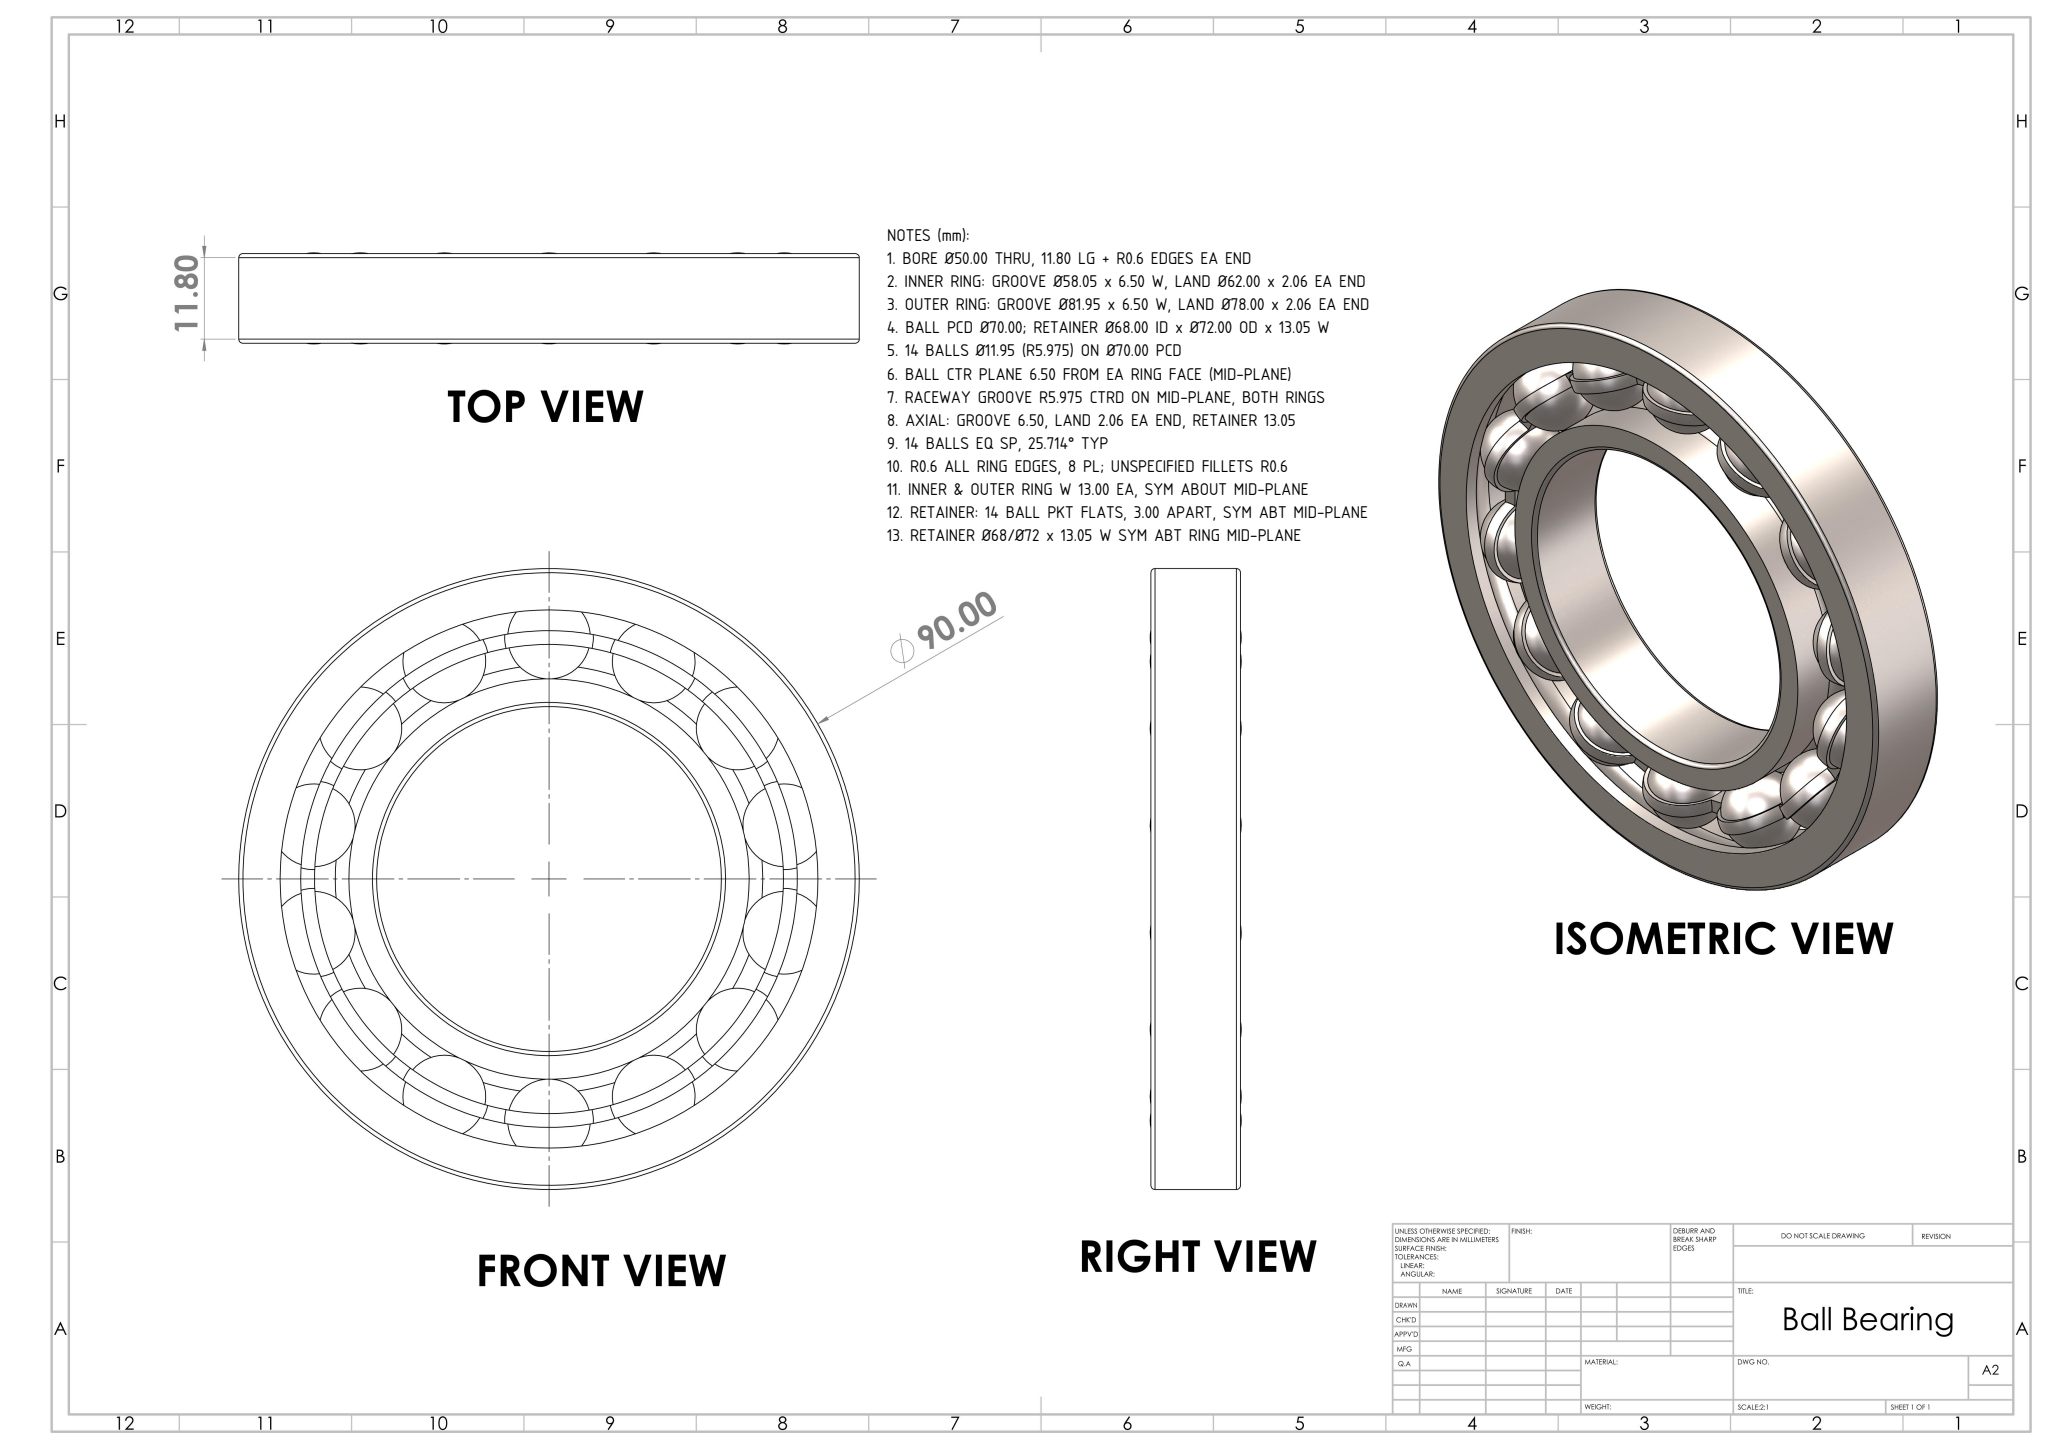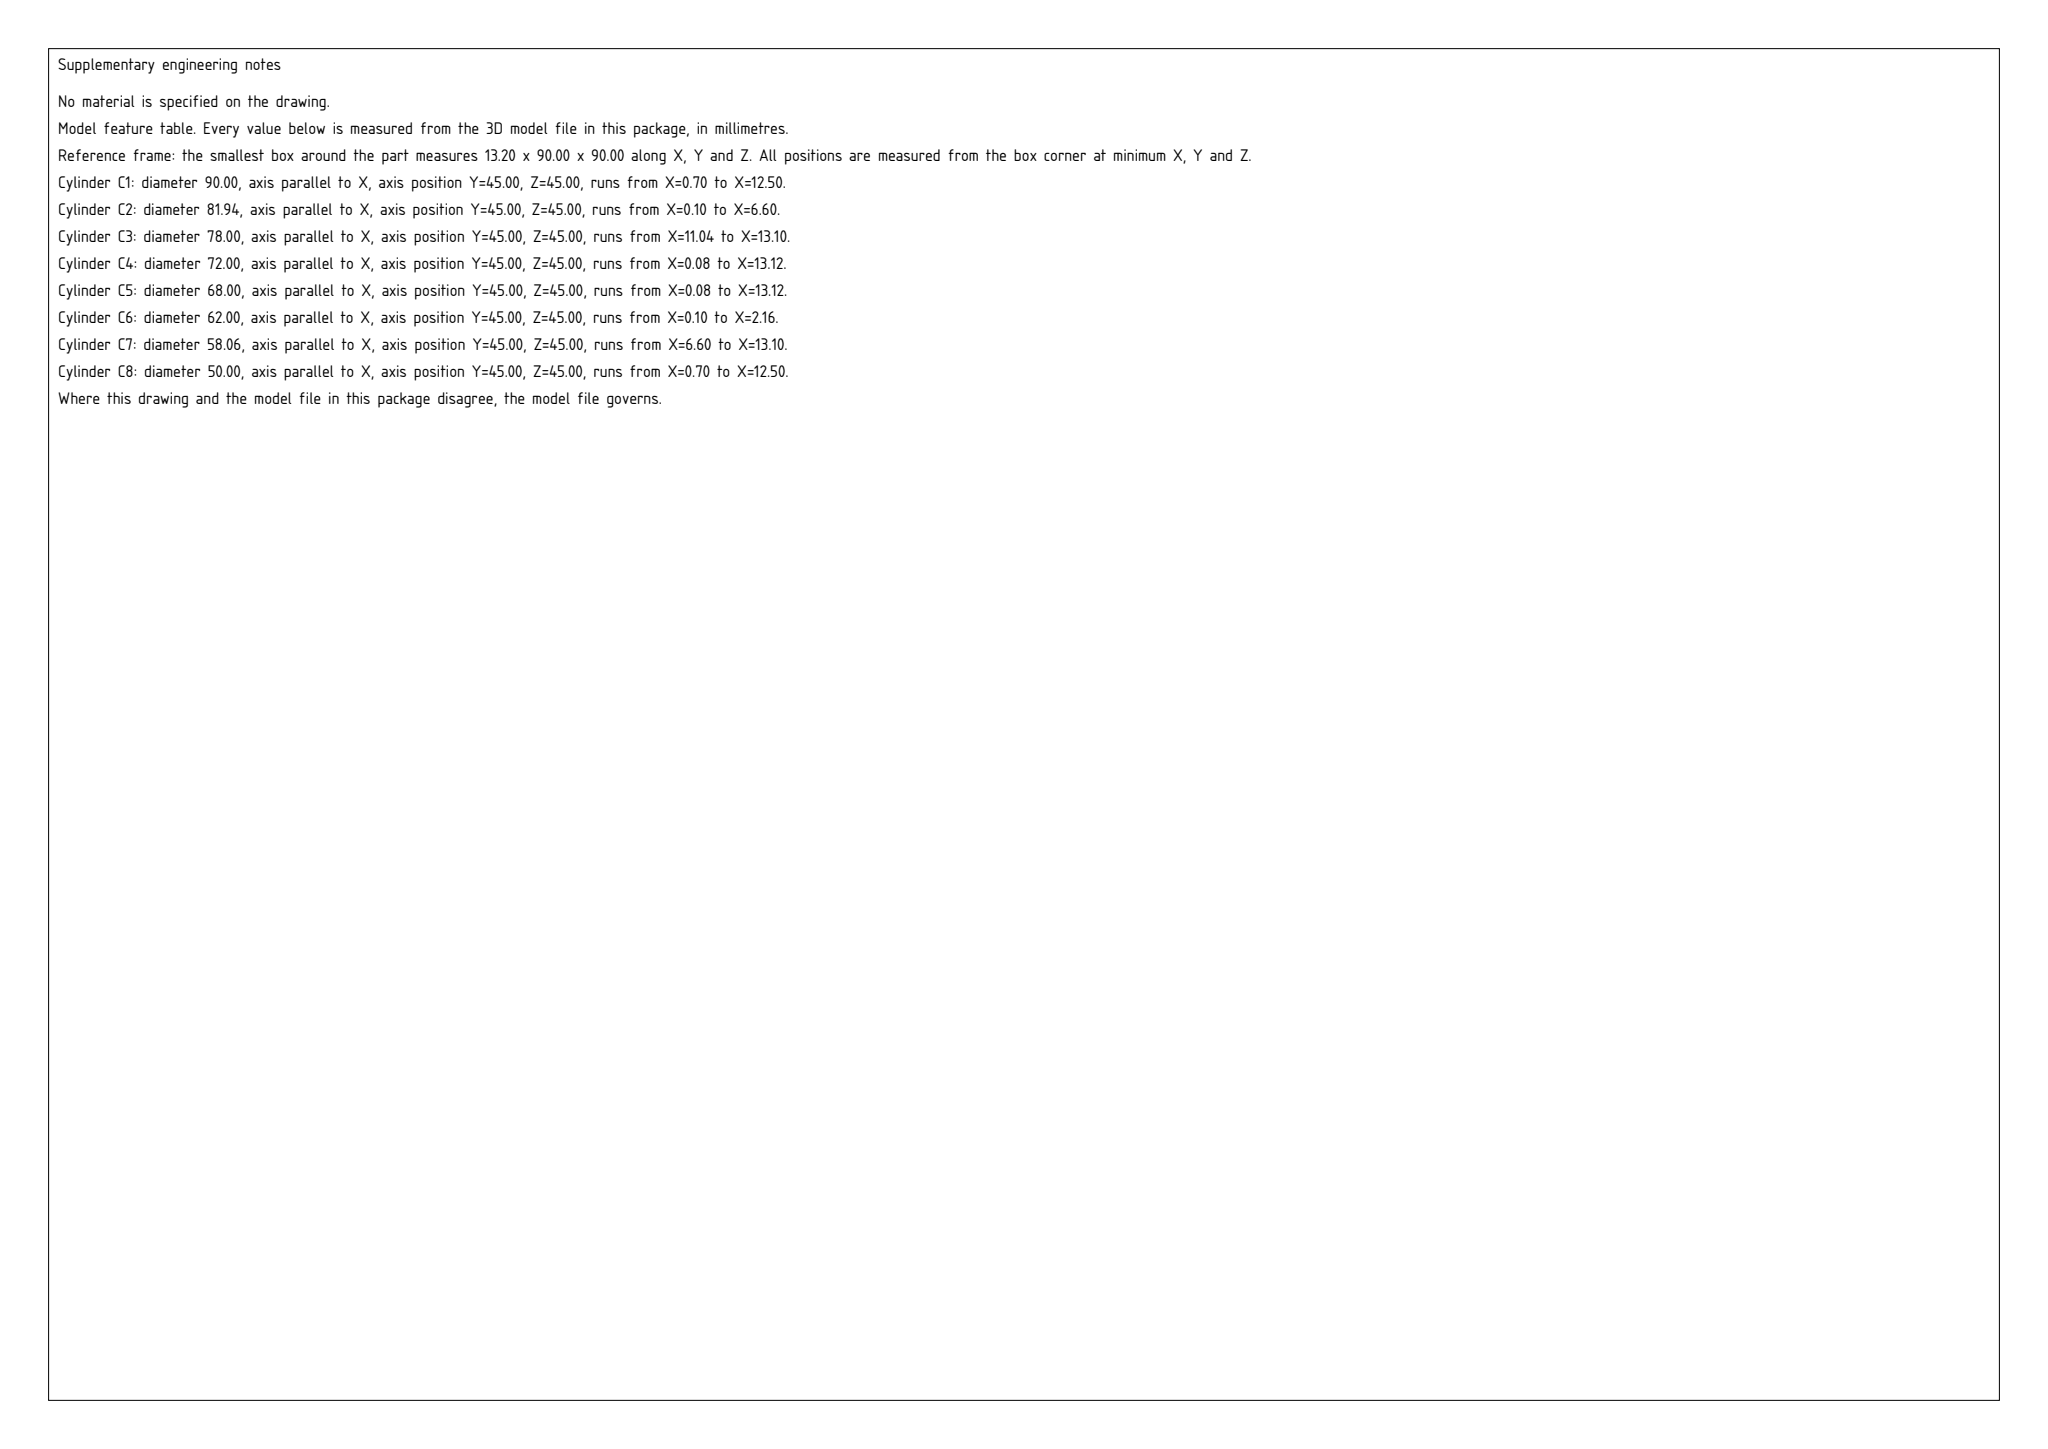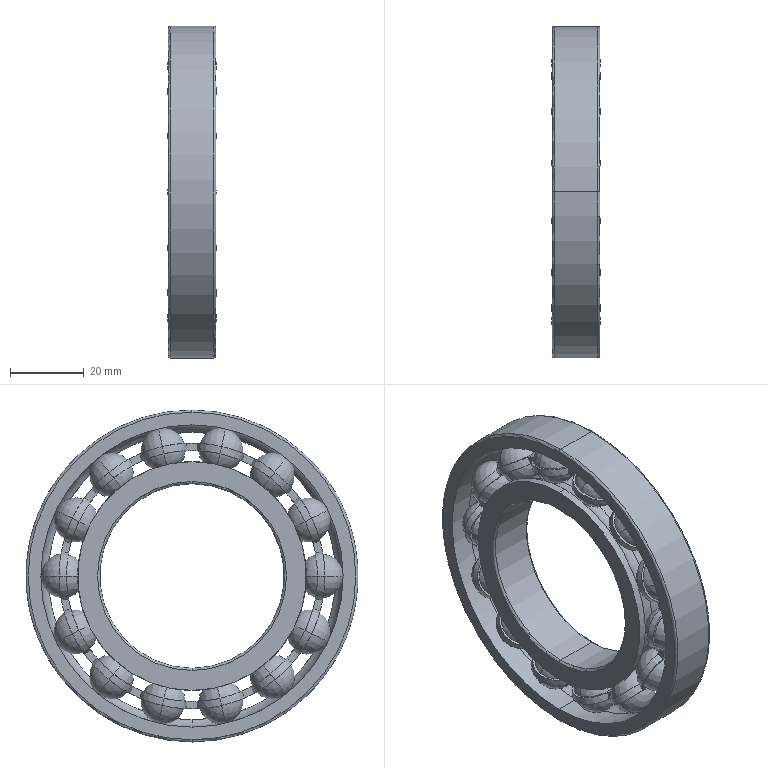Part | SolidWorks | mm | 1 solid | 198 faces | box 13.2 x 90 x 90 mm | volume 39474 mm3 | sphere 112 | torus 38 | plane 32 | cylinder 16 | commonest cylinder face diameters 90 x2 50 x2 62 x2 58.05 x2 68 x2 81.95 x2 78 x2 72 x2
Drawing notes:
BORE Ø50.00 THRU, 11.80 LG + R0.6 EDGES EA END | from the solid: cylinder dia 50.0, axis x, length 11.8 (+2 x R0.6 edge fillets = 13.00 ring width)
INNER RING: GROOVE Ø58.05 x 6.50 W, LAND Ø62.00 x 2.06 EA END | from the solid: cylinders dia 58.05 L6.5 and dia 62.0 L2.06, axis x, centred 48.71,48.71
OUTER RING: GROOVE Ø81.95 x 6.50 W, LAND Ø78.00 x 2.06 EA END | from the solid: cylinders dia 81.95 L6.5 and dia 78.0 L2.06, axis x, centred 48.71,48.71
BALL PCD Ø70.00; RETAINER Ø68.00 ID x Ø72.00 OD x 13.05 W | from the solid: (58.05+81.95)/2=70.00=(68+72)/2; cylinders dia 68.0 & 72.0, L13.05, axis x
14 BALLS Ø11.95 (R5.975) ON Ø70.00 PCD | from the solid: fillet_radii 5.975 x30 = 28 ball faces + 2 raceway grooves; 14 planes at x=5.1/8.1
BALL CTR PLANE 6.50 FROM EA RING FACE (MID-PLANE) | from the solid: ring faces at x=0.1 and x=13.1; mid = 6.6 -> 6.50 from each face
RACEWAY GROOVE R5.975 CTRD ON MID-PLANE, BOTH RINGS | from the solid: fillet_radii 5.975; grooves bottom dia 58.05 / 81.95 symmetric about x=6.6
AXIAL: GROOVE 6.50, LAND 2.06 EA END, RETAINER 13.05 | from the solid: cylinder lengths 6.5 (58.05/81.95), 2.06 (62/78), 13.05 (68/72)
14 BALLS EQ SP, 25.714° TYP | from the solid: 14 planar faces at x=5.1 and 14 at x=8.1; 28 spherical faces R5.975; 360/14
R0.6 ALL RING EDGES, 8 PL; UNSPECIFIED FILLETS R0.6 | from the solid: fillet_radii [0.6, 8]
INNER & OUTER RING W 13.00 EA, SYM ABOUT MID-PLANE | from the solid: x planes at 0.1 (2 faces) and 13.1 (2 faces) => 13.00 width, mid at 6.6
RETAINER: 14 BALL PKT FLATS, 3.00 APART, SYM ABT MID-PLANE | from the solid: axis_planes normal x at offset 5.10 (14) and 8.10 (14); 8.10-5.10=3.00; bbox x=13.2, mid-plane=6.60, 5.10/8.10 sym abt 6.60
RETAINER Ø68/Ø72 x 13.05 W SYM ABT RING MID-PLANE | from the solid: cylinders dia 68.0 and 72.0, axis x, length 13.05 each; centered on bbox x mid-plane 6.60 vs 11.80 W rings